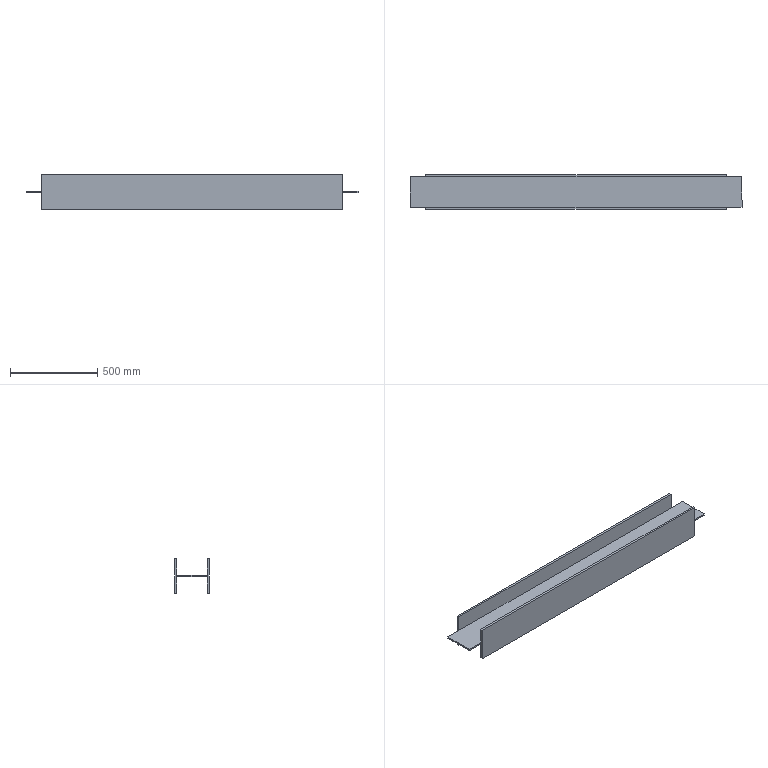Component | SolidWorks | I-Beam200-1905-2 | 1 solid | 22 faces | box 1905 x 200 x 200 mm | volume 10962240 mm3 | plane 22 | material Plain Carbon Steel
build123d program:
from build123d import *

# Parameters (mm, degrees)
BOSS_EXTRUDE1_DEPTH = 1905
SKETCH2_W           = 200
SKETCH2_H           = 90
CUT_EXTRUDE1_DEPTH  = 12
SKETCH3_W           = 200
SKETCH3_H           = 90
CUT_EXTRUDE2_DEPTH  = 12


with BuildPart() as part:
    # Sketch1 → Boss-Extrude1 (new body)
    with BuildSketch(Plane(origin=(0, 0, 0), x_dir=(1, 0, 0), z_dir=(0, 1, 0))):
        Polygon((0, 0), (0, 200), (12, 200), (12, 104), (188, 104), (188, 200), (200, 200), (200, 0), (188, 0), (188, 96), (12, 96), (12, 0), align=None)
    extrude(amount=BOSS_EXTRUDE1_DEPTH)

    # Sketch2 → Cut-Extrude1 (cut)
    with BuildSketch(Plane(origin=(200, 0, 0), x_dir=(0, 0, -1), z_dir=(1, 0, 0))):
        with Locations((100, 1860)):
            Rectangle(SKETCH2_W, SKETCH2_H)
        with Locations((100, 45)):
            Rectangle(SKETCH2_W, SKETCH2_H)
    extrude(amount=-CUT_EXTRUDE1_DEPTH, mode=Mode.SUBTRACT)

    # Sketch3 → Cut-Extrude2 (cut)
    with BuildSketch(Plane.ZY):
        with Locations((-100, 1860)):
            Rectangle(SKETCH3_W, SKETCH3_H)
        with Locations((-100, 45)):
            Rectangle(SKETCH3_W, SKETCH3_H)
    extrude(amount=-CUT_EXTRUDE2_DEPTH, mode=Mode.SUBTRACT)


solid = part.part

# Placed as in the assembly
solid = solid.moved(Location((2489.937, 3009.803, 2380.287), (0, 0, 90)))
STEP:
#1=COLOUR_RGB('',0.7922,0.8196,0.9333);
#2=FILL_AREA_STYLE_COLOUR('',#1);
#3=FILL_AREA_STYLE('',(#2));
#4=SURFACE_STYLE_FILL_AREA(#3);
#5=SURFACE_SIDE_STYLE('',(#4));
#6=SURFACE_STYLE_USAGE(.BOTH.,#5);
#7=PRESENTATION_STYLE_ASSIGNMENT((#6));
#8=CARTESIAN_POINT('',(23.029,118.969,89.933));
#9=VERTEX_POINT('',#8);
#10=CARTESIAN_POINT('',(23.029,118.969,89.618));
#11=VERTEX_POINT('',#10);
#12=CARTESIAN_POINT('',(23.029,118.969,85.838));
#13=DIRECTION('',(0.,0.,-1.));
#14=VECTOR('',#13,39.37);
#15=LINE('',#12,#14);
#16=EDGE_CURVE('',#9,#11,#15,.T.);
#17=ORIENTED_EDGE('',*,*,#16,.F.);
#18=CARTESIAN_POINT('',(23.029,125.898,89.933));
#19=VERTEX_POINT('',#18);
#20=CARTESIAN_POINT('',(23.029,125.898,89.933));
#21=DIRECTION('',(-0.,1.,-0.));
#22=VECTOR('',#21,39.37);
#23=LINE('',#20,#22);
#24=EDGE_CURVE('',#9,#19,#23,.T.);
#25=ORIENTED_EDGE('',*,*,#24,.T.);
#26=CARTESIAN_POINT('',(23.029,125.898,89.618));
#27=VERTEX_POINT('',#26);
#28=CARTESIAN_POINT('',(23.029,125.898,93.712));
#29=DIRECTION('',(-0.,0.,1.));
#30=VECTOR('',#29,39.37);
#31=LINE('',#28,#30);
#32=EDGE_CURVE('',#27,#19,#31,.T.);
#33=ORIENTED_EDGE('',*,*,#32,.F.);
#34=CARTESIAN_POINT('',(23.029,118.969,89.618));
#35=DIRECTION('',(0.,-1.,0.));
#36=VECTOR('',#35,39.37);
#37=LINE('',#34,#36);
#38=EDGE_CURVE('',#27,#11,#37,.T.);
#39=ORIENTED_EDGE('',*,*,#38,.T.);
#40=EDGE_LOOP('',(#17,#25,#33,#39));
#41=FACE_OUTER_BOUND('',#40,.T.);
#42=CARTESIAN_POINT('',(23.029,118.496,93.712));
#43=DIRECTION('',(1.,0.,0.));
#44=DIRECTION('',(0.,0.,-1.));
#45=AXIS2_PLACEMENT_3D('',#42,#43,#44);
#46=PLANE('',#45);
#47=ADVANCED_FACE('',(#41),#46,.F.);
#48=CARTESIAN_POINT('',(98.029,118.969,89.933));
#49=VERTEX_POINT('',#48);
#50=CARTESIAN_POINT('',(98.029,125.898,89.933));
#51=VERTEX_POINT('',#50);
#52=CARTESIAN_POINT('',(98.029,125.898,89.933));
#53=DIRECTION('',(-0.,1.,-0.));
#54=VECTOR('',#53,39.37);
#55=LINE('',#52,#54);
#56=EDGE_CURVE('',#49,#51,#55,.T.);
#57=ORIENTED_EDGE('',*,*,#56,.F.);
#58=CARTESIAN_POINT('',(98.029,118.969,89.618));
#59=VERTEX_POINT('',#58);
#60=CARTESIAN_POINT('',(98.029,118.969,93.712));
#61=DIRECTION('',(0.,0.,1.));
#62=VECTOR('',#61,39.37);
#63=LINE('',#60,#62);
#64=EDGE_CURVE('',#59,#49,#63,.T.);
#65=ORIENTED_EDGE('',*,*,#64,.F.);
#66=CARTESIAN_POINT('',(98.029,125.898,89.618));
#67=VERTEX_POINT('',#66);
#68=CARTESIAN_POINT('',(98.029,118.969,89.618));
#69=DIRECTION('',(0.,-1.,0.));
#70=VECTOR('',#69,39.37);
#71=LINE('',#68,#70);
#72=EDGE_CURVE('',#67,#59,#71,.T.);
#73=ORIENTED_EDGE('',*,*,#72,.F.);
#74=CARTESIAN_POINT('',(98.029,125.898,93.712));
#75=DIRECTION('',(-0.,0.,1.));
#76=VECTOR('',#75,39.37);
#77=LINE('',#74,#76);
#78=EDGE_CURVE('',#67,#51,#77,.T.);
#79=ORIENTED_EDGE('',*,*,#78,.T.);
#80=EDGE_LOOP('',(#57,#65,#73,#79));
#81=FACE_OUTER_BOUND('',#80,.T.);
#82=CARTESIAN_POINT('',(98.029,118.496,93.712));
#83=DIRECTION('',(1.,0.,0.));
#84=DIRECTION('',(0.,0.,-1.));
#85=AXIS2_PLACEMENT_3D('',#82,#83,#84);
#86=PLANE('',#85);
#87=ADVANCED_FACE('',(#81),#86,.T.);
#88=CARTESIAN_POINT('',(26.572,118.969,93.712));
#89=VERTEX_POINT('',#88);
#90=CARTESIAN_POINT('',(94.486,118.969,93.712));
#91=VERTEX_POINT('',#90);
#92=CARTESIAN_POINT('',(23.029,118.969,93.712));
#93=DIRECTION('',(1.,0.,0.));
#94=VECTOR('',#93,39.37);
#95=LINE('',#92,#94);
#96=EDGE_CURVE('',#89,#91,#95,.T.);
#97=ORIENTED_EDGE('',*,*,#96,.F.);
#98=CARTESIAN_POINT('',(26.572,118.496,93.712));
#99=VERTEX_POINT('',#98);
#100=CARTESIAN_POINT('',(26.572,118.969,93.712));
#101=DIRECTION('',(0.,-1.,0.));
#102=VECTOR('',#101,39.37);
#103=LINE('',#100,#102);
#104=EDGE_CURVE('',#89,#99,#103,.T.);
#105=ORIENTED_EDGE('',*,*,#104,.T.);
#106=CARTESIAN_POINT('',(94.486,118.496,93.712));
#107=VERTEX_POINT('',#106);
#108=CARTESIAN_POINT('',(23.029,118.496,93.712));
#109=DIRECTION('',(1.,0.,0.));
#110=VECTOR('',#109,39.37);
#111=LINE('',#108,#110);
#112=EDGE_CURVE('',#99,#107,#111,.T.);
#113=ORIENTED_EDGE('',*,*,#112,.T.);
#114=CARTESIAN_POINT('',(94.486,118.969,93.712));
#115=DIRECTION('',(0.,-1.,0.));
#116=VECTOR('',#115,39.37);
#117=LINE('',#114,#116);
#118=EDGE_CURVE('',#91,#107,#117,.T.);
#119=ORIENTED_EDGE('',*,*,#118,.F.);
#120=EDGE_LOOP('',(#97,#105,#113,#119));
#121=FACE_OUTER_BOUND('',#120,.T.);
#122=CARTESIAN_POINT('',(23.029,118.969,93.712));
#123=DIRECTION('',(-0.,0.,-1.));
#124=DIRECTION('',(0.,-1.,-0.));
#125=AXIS2_PLACEMENT_3D('',#122,#123,#124);
#126=PLANE('',#125);
#127=ADVANCED_FACE('',(#121),#126,.F.);
#128=CARTESIAN_POINT('',(26.572,118.969,89.933));
#129=VERTEX_POINT('',#128);
#130=CARTESIAN_POINT('',(94.486,118.969,89.933));
#131=VERTEX_POINT('',#130);
#132=CARTESIAN_POINT('',(23.029,118.969,89.933));
#133=DIRECTION('',(1.,0.,0.));
#134=VECTOR('',#133,39.37);
#135=LINE('',#132,#134);
#136=EDGE_CURVE('',#129,#131,#135,.T.);
#137=ORIENTED_EDGE('',*,*,#136,.F.);
#138=CARTESIAN_POINT('',(26.572,118.969,85.838));
#139=DIRECTION('',(0.,0.,1.));
#140=VECTOR('',#139,39.37);
#141=LINE('',#138,#140);
#142=EDGE_CURVE('',#129,#89,#141,.T.);
#143=ORIENTED_EDGE('',*,*,#142,.T.);
#144=ORIENTED_EDGE('',*,*,#96,.T.);
#145=CARTESIAN_POINT('',(94.486,118.969,93.712));
#146=DIRECTION('',(0.,0.,-1.));
#147=VECTOR('',#146,39.37);
#148=LINE('',#145,#147);
#149=EDGE_CURVE('',#91,#131,#148,.T.);
#150=ORIENTED_EDGE('',*,*,#149,.T.);
#151=EDGE_LOOP('',(#137,#143,#144,#150));
#152=FACE_OUTER_BOUND('',#151,.T.);
#153=CARTESIAN_POINT('',(23.029,118.969,89.933));
#154=DIRECTION('',(0.,-1.,0.));
#155=DIRECTION('',(-0.,0.,1.));
#156=AXIS2_PLACEMENT_3D('',#153,#154,#155);
#157=PLANE('',#156);
#158=ADVANCED_FACE('',(#152),#157,.F.);
#159=ORIENTED_EDGE('',*,*,#56,.T.);
#160=CARTESIAN_POINT('',(94.486,125.898,89.933));
#161=VERTEX_POINT('',#160);
#162=CARTESIAN_POINT('',(23.029,125.898,89.933));
#163=DIRECTION('',(1.,0.,0.));
#164=VECTOR('',#163,39.37);
#165=LINE('',#162,#164);
#166=EDGE_CURVE('',#161,#51,#165,.T.);
#167=ORIENTED_EDGE('',*,*,#166,.F.);
#168=CARTESIAN_POINT('',(26.572,125.898,89.933));
#169=VERTEX_POINT('',#168);
#170=CARTESIAN_POINT('',(23.029,125.898,89.933));
#171=DIRECTION('',(1.,0.,0.));
#172=VECTOR('',#171,39.37);
#173=LINE('',#170,#172);
#174=EDGE_CURVE('',#169,#161,#173,.T.);
#175=ORIENTED_EDGE('',*,*,#174,.F.);
#176=CARTESIAN_POINT('',(23.029,125.898,89.933));
#177=DIRECTION('',(1.,0.,0.));
#178=VECTOR('',#177,39.37);
#179=LINE('',#176,#178);
#180=EDGE_CURVE('',#19,#169,#179,.T.);
#181=ORIENTED_EDGE('',*,*,#180,.F.);
#182=ORIENTED_EDGE('',*,*,#24,.F.);
#183=CARTESIAN_POINT('',(23.029,118.969,89.933));
#184=DIRECTION('',(1.,0.,0.));
#185=VECTOR('',#184,39.37);
#186=LINE('',#183,#185);
#187=EDGE_CURVE('',#9,#129,#186,.T.);
#188=ORIENTED_EDGE('',*,*,#187,.T.);
#189=ORIENTED_EDGE('',*,*,#136,.T.);
#190=CARTESIAN_POINT('',(23.029,118.969,89.933));
#191=DIRECTION('',(-1.,-0.,0.));
#192=VECTOR('',#191,39.37);
#193=LINE('',#190,#192);
#194=EDGE_CURVE('',#49,#131,#193,.T.);
#195=ORIENTED_EDGE('',*,*,#194,.F.);
#196=EDGE_LOOP('',(#159,#167,#175,#181,#182,#188,#189,#195));
#197=FACE_OUTER_BOUND('',#196,.T.);
#198=CARTESIAN_POINT('',(23.029,125.898,89.933));
#199=DIRECTION('',(0.,-0.,-1.));
#200=DIRECTION('',(0.,-1.,0.));
#201=AXIS2_PLACEMENT_3D('',#198,#199,#200);
#202=PLANE('',#201);
#203=ADVANCED_FACE('',(#197),#202,.F.);
#204=CARTESIAN_POINT('',(26.572,125.898,93.712));
#205=VERTEX_POINT('',#204);
#206=CARTESIAN_POINT('',(94.486,125.898,93.712));
#207=VERTEX_POINT('',#206);
#208=CARTESIAN_POINT('',(23.029,125.898,93.712));
#209=DIRECTION('',(1.,0.,0.));
#210=VECTOR('',#209,39.37);
#211=LINE('',#208,#210);
#212=EDGE_CURVE('',#205,#207,#211,.T.);
#213=ORIENTED_EDGE('',*,*,#212,.F.);
#214=CARTESIAN_POINT('',(26.572,125.898,93.712));
#215=DIRECTION('',(0.,-0.,-1.));
#216=VECTOR('',#215,39.37);
#217=LINE('',#214,#216);
#218=EDGE_CURVE('',#205,#169,#217,.T.);
#219=ORIENTED_EDGE('',*,*,#218,.T.);
#220=ORIENTED_EDGE('',*,*,#174,.T.);
#221=CARTESIAN_POINT('',(94.486,125.898,85.838));
#222=DIRECTION('',(0.,0.,1.));
#223=VECTOR('',#222,39.37);
#224=LINE('',#221,#223);
#225=EDGE_CURVE('',#161,#207,#224,.T.);
#226=ORIENTED_EDGE('',*,*,#225,.T.);
#227=EDGE_LOOP('',(#213,#219,#220,#226));
#228=FACE_OUTER_BOUND('',#227,.T.);
#229=CARTESIAN_POINT('',(23.029,125.898,93.712));
#230=DIRECTION('',(-0.,1.,0.));
#231=DIRECTION('',(-0.,0.,-1.));
#232=AXIS2_PLACEMENT_3D('',#229,#230,#231);
#233=PLANE('',#232);
#234=ADVANCED_FACE('',(#228),#233,.F.);
#235=CARTESIAN_POINT('',(26.572,126.37,93.712));
#236=VERTEX_POINT('',#235);
#237=CARTESIAN_POINT('',(94.486,126.37,93.712));
#238=VERTEX_POINT('',#237);
#239=CARTESIAN_POINT('',(23.029,126.37,93.712));
#240=DIRECTION('',(1.,0.,0.));
#241=VECTOR('',#240,39.37);
#242=LINE('',#239,#241);
#243=EDGE_CURVE('',#236,#238,#242,.T.);
#244=ORIENTED_EDGE('',*,*,#243,.F.);
#245=CARTESIAN_POINT('',(26.572,125.898,93.712));
#246=DIRECTION('',(-0.,1.,-0.));
#247=VECTOR('',#246,39.37);
#248=LINE('',#245,#247);
#249=EDGE_CURVE('',#205,#236,#248,.T.);
#250=ORIENTED_EDGE('',*,*,#249,.F.);
#251=ORIENTED_EDGE('',*,*,#212,.T.);
#252=CARTESIAN_POINT('',(94.486,125.898,93.712));
#253=DIRECTION('',(-0.,1.,-0.));
#254=VECTOR('',#253,39.37);
#255=LINE('',#252,#254);
#256=EDGE_CURVE('',#207,#238,#255,.T.);
#257=ORIENTED_EDGE('',*,*,#256,.T.);
#258=EDGE_LOOP('',(#244,#250,#251,#257));
#259=FACE_OUTER_BOUND('',#258,.T.);
#260=CARTESIAN_POINT('',(23.029,126.37,93.712));
#261=DIRECTION('',(-0.,0.,-1.));
#262=DIRECTION('',(0.,-1.,-0.));
#263=AXIS2_PLACEMENT_3D('',#260,#261,#262);
#264=PLANE('',#263);
#265=ADVANCED_FACE('',(#259),#264,.F.);
#266=CARTESIAN_POINT('',(26.572,126.37,85.838));
#267=VERTEX_POINT('',#266);
#268=CARTESIAN_POINT('',(94.486,126.37,85.838));
#269=VERTEX_POINT('',#268);
#270=CARTESIAN_POINT('',(23.029,126.37,85.838));
#271=DIRECTION('',(1.,0.,0.));
#272=VECTOR('',#271,39.37);
#273=LINE('',#270,#272);
#274=EDGE_CURVE('',#267,#269,#273,.T.);
#275=ORIENTED_EDGE('',*,*,#274,.F.);
#276=CARTESIAN_POINT('',(26.572,126.37,93.712));
#277=DIRECTION('',(0.,-0.,-1.));
#278=VECTOR('',#277,39.37);
#279=LINE('',#276,#278);
#280=EDGE_CURVE('',#236,#267,#279,.T.);
#281=ORIENTED_EDGE('',*,*,#280,.F.);
#282=ORIENTED_EDGE('',*,*,#243,.T.);
#283=CARTESIAN_POINT('',(94.486,126.37,85.838));
#284=DIRECTION('',(0.,0.,1.));
#285=VECTOR('',#284,39.37);
#286=LINE('',#283,#285);
#287=EDGE_CURVE('',#269,#238,#286,.T.);
#288=ORIENTED_EDGE('',*,*,#287,.F.);
#289=EDGE_LOOP('',(#275,#281,#282,#288));
#290=FACE_OUTER_BOUND('',#289,.T.);
#291=CARTESIAN_POINT('',(23.029,126.37,85.838));
#292=DIRECTION('',(0.,-1.,0.));
#293=DIRECTION('',(-0.,0.,1.));
#294=AXIS2_PLACEMENT_3D('',#291,#292,#293);
#295=PLANE('',#294);
#296=ADVANCED_FACE('',(#290),#295,.F.);
#297=CARTESIAN_POINT('',(26.572,125.898,85.838));
#298=VERTEX_POINT('',#297);
#299=CARTESIAN_POINT('',(94.486,125.898,85.838));
#300=VERTEX_POINT('',#299);
#301=CARTESIAN_POINT('',(23.029,125.898,85.838));
#302=DIRECTION('',(1.,0.,0.));
#303=VECTOR('',#302,39.37);
#304=LINE('',#301,#303);
#305=EDGE_CURVE('',#298,#300,#304,.T.);
#306=ORIENTED_EDGE('',*,*,#305,.F.);
#307=CARTESIAN_POINT('',(26.572,125.898,85.838));
#308=DIRECTION('',(-0.,1.,-0.));
#309=VECTOR('',#308,39.37);
#310=LINE('',#307,#309);
#311=EDGE_CURVE('',#298,#267,#310,.T.);
#312=ORIENTED_EDGE('',*,*,#311,.T.);
#313=ORIENTED_EDGE('',*,*,#274,.T.);
#314=CARTESIAN_POINT('',(94.486,125.898,85.838));
#315=DIRECTION('',(-0.,1.,-0.));
#316=VECTOR('',#315,39.37);
#317=LINE('',#314,#316);
#318=EDGE_CURVE('',#300,#269,#317,.T.);
#319=ORIENTED_EDGE('',*,*,#318,.F.);
#320=EDGE_LOOP('',(#306,#312,#313,#319));
#321=FACE_OUTER_BOUND('',#320,.T.);
#322=CARTESIAN_POINT('',(23.029,125.898,85.838));
#323=DIRECTION('',(0.,0.,1.));
#324=DIRECTION('',(-0.,1.,0.));
#325=AXIS2_PLACEMENT_3D('',#322,#323,#324);
#326=PLANE('',#325);
#327=ADVANCED_FACE('',(#321),#326,.F.);
#328=CARTESIAN_POINT('',(26.572,125.898,89.618));
#329=VERTEX_POINT('',#328);
#330=CARTESIAN_POINT('',(94.486,125.898,89.618));
#331=VERTEX_POINT('',#330);
#332=CARTESIAN_POINT('',(23.029,125.898,89.618));
#333=DIRECTION('',(1.,0.,0.));
#334=VECTOR('',#333,39.37);
#335=LINE('',#332,#334);
#336=EDGE_CURVE('',#329,#331,#335,.T.);
#337=ORIENTED_EDGE('',*,*,#336,.F.);
#338=CARTESIAN_POINT('',(26.572,125.898,93.712));
#339=DIRECTION('',(0.,-0.,-1.));
#340=VECTOR('',#339,39.37);
#341=LINE('',#338,#340);
#342=EDGE_CURVE('',#329,#298,#341,.T.);
#343=ORIENTED_EDGE('',*,*,#342,.T.);
#344=ORIENTED_EDGE('',*,*,#305,.T.);
#345=CARTESIAN_POINT('',(94.486,125.898,85.838));
#346=DIRECTION('',(0.,0.,1.));
#347=VECTOR('',#346,39.37);
#348=LINE('',#345,#347);
#349=EDGE_CURVE('',#300,#331,#348,.T.);
#350=ORIENTED_EDGE('',*,*,#349,.T.);
#351=EDGE_LOOP('',(#337,#343,#344,#350));
#352=FACE_OUTER_BOUND('',#351,.T.);
#353=CARTESIAN_POINT('',(23.029,125.898,89.618));
#354=DIRECTION('',(-0.,1.,-0.));
#355=DIRECTION('',(0.,-0.,-1.));
#356=AXIS2_PLACEMENT_3D('',#353,#354,#355);
#357=PLANE('',#356);
#358=ADVANCED_FACE('',(#352),#357,.F.);
#359=ORIENTED_EDGE('',*,*,#72,.T.);
#360=CARTESIAN_POINT('',(94.486,118.969,89.618));
#361=VERTEX_POINT('',#360);
#362=CARTESIAN_POINT('',(23.029,118.969,89.618));
#363=DIRECTION('',(1.,0.,0.));
#364=VECTOR('',#363,39.37);
#365=LINE('',#362,#364);
#366=EDGE_CURVE('',#361,#59,#365,.T.);
#367=ORIENTED_EDGE('',*,*,#366,.F.);
#368=CARTESIAN_POINT('',(26.572,118.969,89.618));
#369=VERTEX_POINT('',#368);
#370=CARTESIAN_POINT('',(23.029,118.969,89.618));
#371=DIRECTION('',(1.,0.,0.));
#372=VECTOR('',#371,39.37);
#373=LINE('',#370,#372);
#374=EDGE_CURVE('',#369,#361,#373,.T.);
#375=ORIENTED_EDGE('',*,*,#374,.F.);
#376=CARTESIAN_POINT('',(23.029,118.969,89.618));
#377=DIRECTION('',(1.,0.,0.));
#378=VECTOR('',#377,39.37);
#379=LINE('',#376,#378);
#380=EDGE_CURVE('',#11,#369,#379,.T.);
#381=ORIENTED_EDGE('',*,*,#380,.F.);
#382=ORIENTED_EDGE('',*,*,#38,.F.);
#383=CARTESIAN_POINT('',(23.029,125.898,89.618));
#384=DIRECTION('',(1.,0.,0.));
#385=VECTOR('',#384,39.37);
#386=LINE('',#383,#385);
#387=EDGE_CURVE('',#27,#329,#386,.T.);
#388=ORIENTED_EDGE('',*,*,#387,.T.);
#389=ORIENTED_EDGE('',*,*,#336,.T.);
#390=CARTESIAN_POINT('',(23.029,125.898,89.618));
#391=DIRECTION('',(-1.,-0.,0.));
#392=VECTOR('',#391,39.37);
#393=LINE('',#390,#392);
#394=EDGE_CURVE('',#67,#331,#393,.T.);
#395=ORIENTED_EDGE('',*,*,#394,.F.);
#396=EDGE_LOOP('',(#359,#367,#375,#381,#382,#388,#389,#395));
#397=FACE_OUTER_BOUND('',#396,.T.);
#398=CARTESIAN_POINT('',(23.029,118.969,89.618));
#399=DIRECTION('',(0.,0.,1.));
#400=DIRECTION('',(-0.,1.,0.));
#401=AXIS2_PLACEMENT_3D('',#398,#399,#400);
#402=PLANE('',#401);
#403=ADVANCED_FACE('',(#397),#402,.F.);
#404=CARTESIAN_POINT('',(26.572,118.969,85.838));
#405=VERTEX_POINT('',#404);
#406=CARTESIAN_POINT('',(94.486,118.969,85.838));
#407=VERTEX_POINT('',#406);
#408=CARTESIAN_POINT('',(23.029,118.969,85.838));
#409=DIRECTION('',(1.,0.,0.));
#410=VECTOR('',#409,39.37);
#411=LINE('',#408,#410);
#412=EDGE_CURVE('',#405,#407,#411,.T.);
#413=ORIENTED_EDGE('',*,*,#412,.F.);
#414=CARTESIAN_POINT('',(26.572,118.969,85.838));
#415=DIRECTION('',(0.,0.,1.));
#416=VECTOR('',#415,39.37);
#417=LINE('',#414,#416);
#418=EDGE_CURVE('',#405,#369,#417,.T.);
#419=ORIENTED_EDGE('',*,*,#418,.T.);
#420=ORIENTED_EDGE('',*,*,#374,.T.);
#421=CARTESIAN_POINT('',(94.486,118.969,93.712));
#422=DIRECTION('',(0.,0.,-1.));
#423=VECTOR('',#422,39.37);
#424=LINE('',#421,#423);
#425=EDGE_CURVE('',#361,#407,#424,.T.);
#426=ORIENTED_EDGE('',*,*,#425,.T.);
#427=EDGE_LOOP('',(#413,#419,#420,#426));
#428=FACE_OUTER_BOUND('',#427,.T.);
#429=CARTESIAN_POINT('',(23.029,118.969,85.838));
#430=DIRECTION('',(0.,-1.,0.));
#431=DIRECTION('',(-0.,0.,1.));
#432=AXIS2_PLACEMENT_3D('',#429,#430,#431);
#433=PLANE('',#432);
#434=ADVANCED_FACE('',(#428),#433,.F.);
#435=CARTESIAN_POINT('',(26.572,118.496,85.838));
#436=VERTEX_POINT('',#435);
#437=CARTESIAN_POINT('',(94.486,118.496,85.838));
#438=VERTEX_POINT('',#437);
#439=CARTESIAN_POINT('',(23.029,118.496,85.838));
#440=DIRECTION('',(1.,0.,0.));
#441=VECTOR('',#440,39.37);
#442=LINE('',#439,#441);
#443=EDGE_CURVE('',#436,#438,#442,.T.);
#444=ORIENTED_EDGE('',*,*,#443,.F.);
#445=CARTESIAN_POINT('',(26.572,118.969,85.838));
#446=DIRECTION('',(0.,-1.,0.));
#447=VECTOR('',#446,39.37);
#448=LINE('',#445,#447);
#449=EDGE_CURVE('',#405,#436,#448,.T.);
#450=ORIENTED_EDGE('',*,*,#449,.F.);
#451=ORIENTED_EDGE('',*,*,#412,.T.);
#452=CARTESIAN_POINT('',(94.486,118.969,85.838));
#453=DIRECTION('',(0.,-1.,0.));
#454=VECTOR('',#453,39.37);
#455=LINE('',#452,#454);
#456=EDGE_CURVE('',#407,#438,#455,.T.);
#457=ORIENTED_EDGE('',*,*,#456,.T.);
#458=EDGE_LOOP('',(#444,#450,#451,#457));
#459=FACE_OUTER_BOUND('',#458,.T.);
#460=CARTESIAN_POINT('',(23.029,118.496,85.838));
#461=DIRECTION('',(0.,0.,1.));
#462=DIRECTION('',(-0.,1.,0.));
#463=AXIS2_PLACEMENT_3D('',#460,#461,#462);
#464=PLANE('',#463);
#465=ADVANCED_FACE('',(#459),#464,.F.);
#466=ORIENTED_EDGE('',*,*,#112,.F.);
#467=CARTESIAN_POINT('',(26.572,118.496,85.838));
#468=DIRECTION('',(0.,0.,1.));
#469=VECTOR('',#468,39.37);
#470=LINE('',#467,#469);
#471=EDGE_CURVE('',#436,#99,#470,.T.);
#472=ORIENTED_EDGE('',*,*,#471,.F.);
#473=ORIENTED_EDGE('',*,*,#443,.T.);
#474=CARTESIAN_POINT('',(94.486,118.496,93.712));
#475=DIRECTION('',(0.,0.,-1.));
#476=VECTOR('',#475,39.37);
#477=LINE('',#474,#476);
#478=EDGE_CURVE('',#107,#438,#477,.T.);
#479=ORIENTED_EDGE('',*,*,#478,.F.);
#480=EDGE_LOOP('',(#466,#472,#473,#479));
#481=FACE_OUTER_BOUND('',#480,.T.);
#482=CARTESIAN_POINT('',(23.029,118.496,93.712));
#483=DIRECTION('',(-0.,1.,0.));
#484=DIRECTION('',(0.,0.,-1.));
#485=AXIS2_PLACEMENT_3D('',#482,#483,#484);
#486=PLANE('',#485);
#487=ADVANCED_FACE('',(#481),#486,.F.);
#488=ORIENTED_EDGE('',*,*,#166,.T.);
#489=ORIENTED_EDGE('',*,*,#78,.F.);
#490=ORIENTED_EDGE('',*,*,#394,.T.);
#491=CARTESIAN_POINT('',(94.486,125.898,85.838));
#492=DIRECTION('',(0.,0.,1.));
#493=VECTOR('',#492,39.37);
#494=LINE('',#491,#493);
#495=EDGE_CURVE('',#331,#161,#494,.T.);
#496=ORIENTED_EDGE('',*,*,#495,.T.);
#497=EDGE_LOOP('',(#488,#489,#490,#496));
#498=FACE_OUTER_BOUND('',#497,.T.);
#499=CARTESIAN_POINT('',(98.029,125.898,93.712));
#500=DIRECTION('',(-0.,1.,-0.));
#501=DIRECTION('',(0.,-0.,-1.));
#502=AXIS2_PLACEMENT_3D('',#499,#500,#501);
#503=PLANE('',#502);
#504=ADVANCED_FACE('',(#498),#503,.T.);
#505=ORIENTED_EDGE('',*,*,#287,.T.);
#506=ORIENTED_EDGE('',*,*,#256,.F.);
#507=ORIENTED_EDGE('',*,*,#225,.F.);
#508=ORIENTED_EDGE('',*,*,#495,.F.);
#509=ORIENTED_EDGE('',*,*,#349,.F.);
#510=ORIENTED_EDGE('',*,*,#318,.T.);
#511=EDGE_LOOP('',(#505,#506,#507,#508,#509,#510));
#512=FACE_OUTER_BOUND('',#511,.T.);
#513=CARTESIAN_POINT('',(94.486,125.898,85.838));
#514=DIRECTION('',(-1.,-0.,0.));
#515=DIRECTION('',(0.,0.,1.));
#516=AXIS2_PLACEMENT_3D('',#513,#514,#515);
#517=PLANE('',#516);
#518=ADVANCED_FACE('',(#512),#517,.F.);
#519=ORIENTED_EDGE('',*,*,#180,.T.);
#520=CARTESIAN_POINT('',(26.572,125.898,93.712));
#521=DIRECTION('',(0.,-0.,-1.));
#522=VECTOR('',#521,39.37);
#523=LINE('',#520,#522);
#524=EDGE_CURVE('',#169,#329,#523,.T.);
#525=ORIENTED_EDGE('',*,*,#524,.T.);
#526=ORIENTED_EDGE('',*,*,#387,.F.);
#527=ORIENTED_EDGE('',*,*,#32,.T.);
#528=EDGE_LOOP('',(#519,#525,#526,#527));
#529=FACE_OUTER_BOUND('',#528,.T.);
#530=CARTESIAN_POINT('',(98.029,125.898,93.712));
#531=DIRECTION('',(-0.,1.,-0.));
#532=DIRECTION('',(0.,-0.,-1.));
#533=AXIS2_PLACEMENT_3D('',#530,#531,#532);
#534=PLANE('',#533);
#535=ADVANCED_FACE('',(#529),#534,.T.);
#536=ORIENTED_EDGE('',*,*,#280,.T.);
#537=ORIENTED_EDGE('',*,*,#311,.F.);
#538=ORIENTED_EDGE('',*,*,#342,.F.);
#539=ORIENTED_EDGE('',*,*,#524,.F.);
#540=ORIENTED_EDGE('',*,*,#218,.F.);
#541=ORIENTED_EDGE('',*,*,#249,.T.);
#542=EDGE_LOOP('',(#536,#537,#538,#539,#540,#541));
#543=FACE_OUTER_BOUND('',#542,.T.);
#544=CARTESIAN_POINT('',(26.572,125.898,93.712));
#545=DIRECTION('',(1.,0.,0.));
#546=DIRECTION('',(0.,0.,-1.));
#547=AXIS2_PLACEMENT_3D('',#544,#545,#546);
#548=PLANE('',#547);
#549=ADVANCED_FACE('',(#543),#548,.F.);
#550=ORIENTED_EDGE('',*,*,#194,.T.);
#551=CARTESIAN_POINT('',(94.486,118.969,93.712));
#552=DIRECTION('',(0.,0.,-1.));
#553=VECTOR('',#552,39.37);
#554=LINE('',#551,#553);
#555=EDGE_CURVE('',#131,#361,#554,.T.);
#556=ORIENTED_EDGE('',*,*,#555,.T.);
#557=ORIENTED_EDGE('',*,*,#366,.T.);
#558=ORIENTED_EDGE('',*,*,#64,.T.);
#559=EDGE_LOOP('',(#550,#556,#557,#558));
#560=FACE_OUTER_BOUND('',#559,.T.);
#561=CARTESIAN_POINT('',(98.029,118.969,93.712));
#562=DIRECTION('',(0.,-1.,0.));
#563=DIRECTION('',(0.,0.,1.));
#564=AXIS2_PLACEMENT_3D('',#561,#562,#563);
#565=PLANE('',#564);
#566=ADVANCED_FACE('',(#560),#565,.T.);
#567=ORIENTED_EDGE('',*,*,#478,.T.);
#568=ORIENTED_EDGE('',*,*,#456,.F.);
#569=ORIENTED_EDGE('',*,*,#425,.F.);
#570=ORIENTED_EDGE('',*,*,#555,.F.);
#571=ORIENTED_EDGE('',*,*,#149,.F.);
#572=ORIENTED_EDGE('',*,*,#118,.T.);
#573=EDGE_LOOP('',(#567,#568,#569,#570,#571,#572));
#574=FACE_OUTER_BOUND('',#573,.T.);
#575=CARTESIAN_POINT('',(94.486,118.969,93.712));
#576=DIRECTION('',(-1.,-0.,-0.));
#577=DIRECTION('',(-0.,-0.,1.));
#578=AXIS2_PLACEMENT_3D('',#575,#576,#577);
#579=PLANE('',#578);
#580=ADVANCED_FACE('',(#574),#579,.F.);
#581=ORIENTED_EDGE('',*,*,#187,.F.);
#582=ORIENTED_EDGE('',*,*,#16,.T.);
#583=ORIENTED_EDGE('',*,*,#380,.T.);
#584=CARTESIAN_POINT('',(26.572,118.969,85.838));
#585=DIRECTION('',(0.,0.,1.));
#586=VECTOR('',#585,39.37);
#587=LINE('',#584,#586);
#588=EDGE_CURVE('',#369,#129,#587,.T.);
#589=ORIENTED_EDGE('',*,*,#588,.T.);
#590=EDGE_LOOP('',(#581,#582,#583,#589));
#591=FACE_OUTER_BOUND('',#590,.T.);
#592=CARTESIAN_POINT('',(98.029,118.969,93.712));
#593=DIRECTION('',(0.,-1.,0.));
#594=DIRECTION('',(0.,0.,1.));
#595=AXIS2_PLACEMENT_3D('',#592,#593,#594);
#596=PLANE('',#595);
#597=ADVANCED_FACE('',(#591),#596,.T.);
#598=ORIENTED_EDGE('',*,*,#471,.T.);
#599=ORIENTED_EDGE('',*,*,#104,.F.);
#600=ORIENTED_EDGE('',*,*,#142,.F.);
#601=ORIENTED_EDGE('',*,*,#588,.F.);
#602=ORIENTED_EDGE('',*,*,#418,.F.);
#603=ORIENTED_EDGE('',*,*,#449,.T.);
#604=EDGE_LOOP('',(#598,#599,#600,#601,#602,#603));
#605=FACE_OUTER_BOUND('',#604,.T.);
#606=CARTESIAN_POINT('',(26.572,118.969,85.838));
#607=DIRECTION('',(1.,0.,0.));
#608=DIRECTION('',(0.,0.,-1.));
#609=AXIS2_PLACEMENT_3D('',#606,#607,#608);
#610=PLANE('',#609);
#611=ADVANCED_FACE('',(#605),#610,.F.);
#612=CLOSED_SHELL('',(#47,#87,#127,#158,#203,#234,#265,#296,#327,#358,#403,#434,#465,#487,#504,#518,#535,#549,#566,#580,#597,#611));
#613=MANIFOLD_SOLID_BREP('',#612);
#614=STYLED_ITEM('',(#7),#613);
#615=(LENGTH_UNIT()NAMED_UNIT(*)SI_UNIT($,.METRE.));
#616=LENGTH_MEASURE_WITH_UNIT(LENGTH_MEASURE(0.0254),#615);
#617=DIMENSIONAL_EXPONENTS(1.,0.,0.,0.,0.,0.,0.);
#618=(CONVERSION_BASED_UNIT('',#616)LENGTH_UNIT()NAMED_UNIT(#617));
#619=UNCERTAINTY_MEASURE_WITH_UNIT(LENGTH_MEASURE(0.00001),#618,'','');
#620=(NAMED_UNIT(*)PLANE_ANGLE_UNIT()SI_UNIT($,.RADIAN.));
#621=(NAMED_UNIT(*)SI_UNIT($,.STERADIAN.)SOLID_ANGLE_UNIT());
#622=(GEOMETRIC_REPRESENTATION_CONTEXT(3)GLOBAL_UNCERTAINTY_ASSIGNED_CONTEXT((#619))GLOBAL_UNIT_ASSIGNED_CONTEXT((#618,#620,#621))REPRESENTATION_CONTEXT('',''));
#623=MECHANICAL_DESIGN_GEOMETRIC_PRESENTATION_REPRESENTATION('',(#614),#622);
#624=PRESENTATION_LAYER_ASSIGNMENT('','',(#614));
#625=CARTESIAN_POINT('',(0.,0.,0.));
#626=DIRECTION('',(0.,0.,1.));
#627=DIRECTION('',(1.,0.,0.));
#628=AXIS2_PLACEMENT_3D('',#625,#626,#627);
#629=(LENGTH_UNIT()NAMED_UNIT(*)SI_UNIT($,.METRE.));
#630=LENGTH_MEASURE_WITH_UNIT(LENGTH_MEASURE(0.0254),#629);
#631=DIMENSIONAL_EXPONENTS(1.,0.,0.,0.,0.,0.,0.);
#632=(CONVERSION_BASED_UNIT('',#630)LENGTH_UNIT()NAMED_UNIT(#631));
#633=UNCERTAINTY_MEASURE_WITH_UNIT(LENGTH_MEASURE(0.00001),#632,'','');
#634=(NAMED_UNIT(*)PLANE_ANGLE_UNIT()SI_UNIT($,.RADIAN.));
#635=(NAMED_UNIT(*)SI_UNIT($,.STERADIAN.)SOLID_ANGLE_UNIT());
#636=(GEOMETRIC_REPRESENTATION_CONTEXT(3)GLOBAL_UNCERTAINTY_ASSIGNED_CONTEXT((#633))GLOBAL_UNIT_ASSIGNED_CONTEXT((#632,#634,#635))REPRESENTATION_CONTEXT('',''));
#637=ADVANCED_BREP_SHAPE_REPRESENTATION('',(#613,#628),#636);